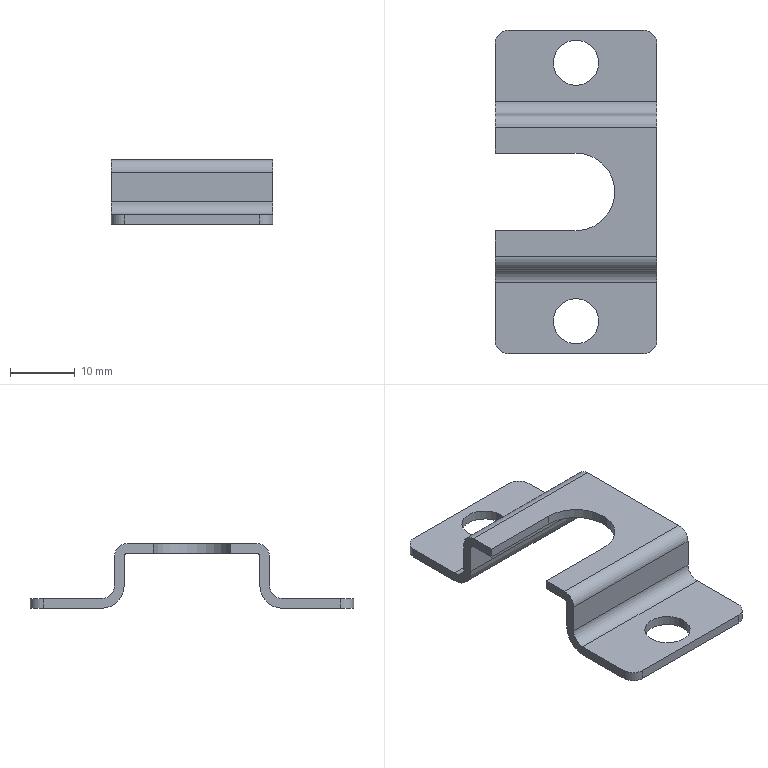Component | SolidWorks | DirectPressureVerticalSeal-1_Fastener-1 | 1 solid | 34 faces | box 25 x 50 x 10 mm | volume 1953 mm3 | cylinder 17 | plane 17 | commonest cylinder face diameters 4 x8 7 x6 1 x2 12 x1
STEP:
#1=CARTESIAN_POINT('',(-11.899,10.507,10.002));
#2=VERTEX_POINT('',#1);
#3=CARTESIAN_POINT('',(-11.624,10.507,10.002));
#4=VERTEX_POINT('',#3);
#5=CARTESIAN_POINT('',(-11.762,10.507,10.002));
#6=DIRECTION('',(-0.,0.,1.));
#7=DIRECTION('',(1.,0.,0.));
#8=AXIS2_PLACEMENT_3D('',#5,#6,#7);
#9=CIRCLE('',#8,0.1378);
#10=EDGE_CURVE('',#2,#4,#9,.T.);
#11=ORIENTED_EDGE('',*,*,#10,.F.);
#12=CARTESIAN_POINT('',(-11.899,10.507,10.061));
#13=VERTEX_POINT('',#12);
#14=CARTESIAN_POINT('',(-11.899,10.507,10.061));
#15=DIRECTION('',(-0.,0.,1.));
#16=VECTOR('',#15,39.37);
#17=LINE('',#14,#16);
#18=EDGE_CURVE('',#2,#13,#17,.T.);
#19=ORIENTED_EDGE('',*,*,#18,.T.);
#20=CARTESIAN_POINT('',(-11.624,10.507,10.061));
#21=VERTEX_POINT('',#20);
#22=CARTESIAN_POINT('',(-11.762,10.507,10.061));
#23=DIRECTION('',(-0.,0.,1.));
#24=DIRECTION('',(1.,0.,0.));
#25=AXIS2_PLACEMENT_3D('',#22,#23,#24);
#26=CIRCLE('',#25,0.1378);
#27=EDGE_CURVE('',#13,#21,#26,.T.);
#28=ORIENTED_EDGE('',*,*,#27,.T.);
#29=CARTESIAN_POINT('',(-11.624,10.507,10.061));
#30=DIRECTION('',(-0.,0.,1.));
#31=VECTOR('',#30,39.37);
#32=LINE('',#29,#31);
#33=EDGE_CURVE('',#4,#21,#32,.T.);
#34=ORIENTED_EDGE('',*,*,#33,.F.);
#35=EDGE_LOOP('',(#11,#19,#28,#34));
#36=FACE_OUTER_BOUND('',#35,.T.);
#37=CARTESIAN_POINT('',(-11.762,10.507,10.061));
#38=DIRECTION('',(-0.,0.,1.));
#39=DIRECTION('',(1.,0.,0.));
#40=AXIS2_PLACEMENT_3D('',#37,#38,#39);
#41=CYLINDRICAL_SURFACE('',#40,0.1378);
#42=ADVANCED_FACE('',(#36),#41,.F.);
#43=CARTESIAN_POINT('',(-11.624,8.932,10.061));
#44=VERTEX_POINT('',#43);
#45=CARTESIAN_POINT('',(-11.899,8.932,10.061));
#46=VERTEX_POINT('',#45);
#47=CARTESIAN_POINT('',(-11.762,8.932,10.061));
#48=DIRECTION('',(0.,-0.,-1.));
#49=DIRECTION('',(0.,1.,0.));
#50=AXIS2_PLACEMENT_3D('',#47,#48,#49);
#51=CIRCLE('',#50,0.1378);
#52=EDGE_CURVE('',#44,#46,#51,.T.);
#53=ORIENTED_EDGE('',*,*,#52,.F.);
#54=CARTESIAN_POINT('',(-11.624,8.932,10.002));
#55=VERTEX_POINT('',#54);
#56=CARTESIAN_POINT('',(-11.624,8.932,10.002));
#57=DIRECTION('',(0.,-0.,-1.));
#58=VECTOR('',#57,39.37);
#59=LINE('',#56,#58);
#60=EDGE_CURVE('',#44,#55,#59,.T.);
#61=ORIENTED_EDGE('',*,*,#60,.T.);
#62=CARTESIAN_POINT('',(-11.899,8.932,10.002));
#63=VERTEX_POINT('',#62);
#64=CARTESIAN_POINT('',(-11.762,8.932,10.002));
#65=DIRECTION('',(0.,-0.,-1.));
#66=DIRECTION('',(-1.,0.,0.));
#67=AXIS2_PLACEMENT_3D('',#64,#65,#66);
#68=CIRCLE('',#67,0.1378);
#69=EDGE_CURVE('',#55,#63,#68,.T.);
#70=ORIENTED_EDGE('',*,*,#69,.T.);
#71=CARTESIAN_POINT('',(-11.899,8.932,10.002));
#72=DIRECTION('',(0.,-0.,-1.));
#73=VECTOR('',#72,39.37);
#74=LINE('',#71,#73);
#75=EDGE_CURVE('',#46,#63,#74,.T.);
#76=ORIENTED_EDGE('',*,*,#75,.F.);
#77=EDGE_LOOP('',(#53,#61,#70,#76));
#78=FACE_OUTER_BOUND('',#77,.T.);
#79=CARTESIAN_POINT('',(-11.762,8.932,10.002));
#80=DIRECTION('',(0.,-0.,-1.));
#81=DIRECTION('',(-1.,0.,0.));
#82=AXIS2_PLACEMENT_3D('',#79,#80,#81);
#83=CYLINDRICAL_SURFACE('',#82,0.1378);
#84=ADVANCED_FACE('',(#78),#83,.F.);
#85=CARTESIAN_POINT('',(-12.254,9.956,10.337));
#86=VERTEX_POINT('',#85);
#87=CARTESIAN_POINT('',(-12.254,10.113,10.337));
#88=VERTEX_POINT('',#87);
#89=CARTESIAN_POINT('',(-12.254,9.168,10.337));
#90=DIRECTION('',(-0.,1.,-0.));
#91=VECTOR('',#90,39.37);
#92=LINE('',#89,#91);
#93=EDGE_CURVE('',#86,#88,#92,.T.);
#94=ORIENTED_EDGE('',*,*,#93,.F.);
#95=CARTESIAN_POINT('',(-12.254,9.956,10.396));
#96=VERTEX_POINT('',#95);
#97=CARTESIAN_POINT('',(-12.254,9.956,10.002));
#98=DIRECTION('',(-0.,0.,1.));
#99=VECTOR('',#98,39.37);
#100=LINE('',#97,#99);
#101=EDGE_CURVE('',#86,#96,#100,.T.);
#102=ORIENTED_EDGE('',*,*,#101,.T.);
#103=CARTESIAN_POINT('',(-12.254,10.113,10.396));
#104=VERTEX_POINT('',#103);
#105=CARTESIAN_POINT('',(-12.254,10.113,10.396));
#106=DIRECTION('',(-0.,1.,-0.));
#107=VECTOR('',#106,39.37);
#108=LINE('',#105,#107);
#109=EDGE_CURVE('',#96,#104,#108,.T.);
#110=ORIENTED_EDGE('',*,*,#109,.T.);
#111=CARTESIAN_POINT('',(-12.254,10.192,10.317));
#112=VERTEX_POINT('',#111);
#113=CARTESIAN_POINT('',(-12.254,10.113,10.317));
#114=DIRECTION('',(1.,0.,0.));
#115=DIRECTION('',(0.,0.,1.));
#116=AXIS2_PLACEMENT_3D('',#113,#114,#115);
#117=CIRCLE('',#116,0.07874);
#118=EDGE_CURVE('',#112,#104,#117,.T.);
#119=ORIENTED_EDGE('',*,*,#118,.F.);
#120=CARTESIAN_POINT('',(-12.254,10.192,10.14));
#121=VERTEX_POINT('',#120);
#122=CARTESIAN_POINT('',(-12.254,10.192,10.14));
#123=DIRECTION('',(-0.,0.,1.));
#124=VECTOR('',#123,39.37);
#125=LINE('',#122,#124);
#126=EDGE_CURVE('',#121,#112,#125,.T.);
#127=ORIENTED_EDGE('',*,*,#126,.F.);
#128=CARTESIAN_POINT('',(-12.254,10.271,10.061));
#129=VERTEX_POINT('',#128);
#130=CARTESIAN_POINT('',(-12.254,10.271,10.14));
#131=DIRECTION('',(-1.,-0.,-0.));
#132=DIRECTION('',(0.,0.,1.));
#133=AXIS2_PLACEMENT_3D('',#130,#131,#132);
#134=CIRCLE('',#133,0.07874);
#135=EDGE_CURVE('',#129,#121,#134,.T.);
#136=ORIENTED_EDGE('',*,*,#135,.F.);
#137=CARTESIAN_POINT('',(-12.254,10.625,10.061));
#138=VERTEX_POINT('',#137);
#139=CARTESIAN_POINT('',(-12.254,9.168,10.061));
#140=DIRECTION('',(0.,-1.,0.));
#141=VECTOR('',#140,39.37);
#142=LINE('',#139,#141);
#143=EDGE_CURVE('',#138,#129,#142,.T.);
#144=ORIENTED_EDGE('',*,*,#143,.F.);
#145=CARTESIAN_POINT('',(-12.254,10.625,10.002));
#146=VERTEX_POINT('',#145);
#147=CARTESIAN_POINT('',(-12.254,10.625,10.14));
#148=DIRECTION('',(-0.,0.,1.));
#149=VECTOR('',#148,39.37);
#150=LINE('',#147,#149);
#151=EDGE_CURVE('',#146,#138,#150,.T.);
#152=ORIENTED_EDGE('',*,*,#151,.F.);
#153=CARTESIAN_POINT('',(-12.254,10.271,10.002));
#154=VERTEX_POINT('',#153);
#155=CARTESIAN_POINT('',(-12.254,9.168,10.002));
#156=DIRECTION('',(-0.,1.,-0.));
#157=VECTOR('',#156,39.37);
#158=LINE('',#155,#157);
#159=EDGE_CURVE('',#154,#146,#158,.T.);
#160=ORIENTED_EDGE('',*,*,#159,.F.);
#161=CARTESIAN_POINT('',(-12.254,10.133,10.14));
#162=VERTEX_POINT('',#161);
#163=CARTESIAN_POINT('',(-12.254,10.271,10.14));
#164=DIRECTION('',(1.,0.,0.));
#165=DIRECTION('',(0.,0.,1.));
#166=AXIS2_PLACEMENT_3D('',#163,#164,#165);
#167=CIRCLE('',#166,0.1378);
#168=EDGE_CURVE('',#162,#154,#167,.T.);
#169=ORIENTED_EDGE('',*,*,#168,.F.);
#170=CARTESIAN_POINT('',(-12.254,10.133,10.317));
#171=VERTEX_POINT('',#170);
#172=CARTESIAN_POINT('',(-12.254,10.133,10.14));
#173=DIRECTION('',(0.,-0.,-1.));
#174=VECTOR('',#173,39.37);
#175=LINE('',#172,#174);
#176=EDGE_CURVE('',#171,#162,#175,.T.);
#177=ORIENTED_EDGE('',*,*,#176,.F.);
#178=CARTESIAN_POINT('',(-12.254,10.113,10.317));
#179=DIRECTION('',(1.,0.,0.));
#180=DIRECTION('',(0.,0.,1.));
#181=AXIS2_PLACEMENT_3D('',#178,#179,#180);
#182=CIRCLE('',#181,0.01969);
#183=EDGE_CURVE('',#171,#88,#182,.T.);
#184=ORIENTED_EDGE('',*,*,#183,.T.);
#185=EDGE_LOOP('',(#94,#102,#110,#119,#127,#136,#144,#152,#160,#169,#177,#184));
#186=FACE_OUTER_BOUND('',#185,.T.);
#187=CARTESIAN_POINT('',(-12.254,9.168,10.14));
#188=DIRECTION('',(1.,0.,0.));
#189=DIRECTION('',(0.,-0.,-1.));
#190=AXIS2_PLACEMENT_3D('',#187,#188,#189);
#191=PLANE('',#190);
#192=ADVANCED_FACE('',(#186),#191,.F.);
#193=ORIENTED_EDGE('',*,*,#109,.F.);
#194=CARTESIAN_POINT('',(-11.762,9.956,10.396));
#195=VERTEX_POINT('',#194);
#196=CARTESIAN_POINT('',(-11.762,9.956,10.396));
#197=DIRECTION('',(-1.,-0.,-0.));
#198=VECTOR('',#197,39.37);
#199=LINE('',#196,#198);
#200=EDGE_CURVE('',#195,#96,#199,.T.);
#201=ORIENTED_EDGE('',*,*,#200,.F.);
#202=CARTESIAN_POINT('',(-11.762,9.483,10.396));
#203=VERTEX_POINT('',#202);
#204=CARTESIAN_POINT('',(-11.762,9.719,10.396));
#205=DIRECTION('',(-0.,0.,1.));
#206=DIRECTION('',(0.,-1.,0.));
#207=AXIS2_PLACEMENT_3D('',#204,#205,#206);
#208=CIRCLE('',#207,0.2362);
#209=EDGE_CURVE('',#203,#195,#208,.T.);
#210=ORIENTED_EDGE('',*,*,#209,.F.);
#211=CARTESIAN_POINT('',(-12.254,9.483,10.396));
#212=VERTEX_POINT('',#211);
#213=CARTESIAN_POINT('',(-12.254,9.483,10.396));
#214=DIRECTION('',(1.,0.,0.));
#215=VECTOR('',#214,39.37);
#216=LINE('',#213,#215);
#217=EDGE_CURVE('',#212,#203,#216,.T.);
#218=ORIENTED_EDGE('',*,*,#217,.F.);
#219=CARTESIAN_POINT('',(-12.254,9.326,10.396));
#220=VERTEX_POINT('',#219);
#221=CARTESIAN_POINT('',(-12.254,10.113,10.396));
#222=DIRECTION('',(-0.,1.,-0.));
#223=VECTOR('',#222,39.37);
#224=LINE('',#221,#223);
#225=EDGE_CURVE('',#220,#212,#224,.T.);
#226=ORIENTED_EDGE('',*,*,#225,.F.);
#227=CARTESIAN_POINT('',(-11.27,9.326,10.396));
#228=VERTEX_POINT('',#227);
#229=CARTESIAN_POINT('',(-11.27,9.326,10.396));
#230=DIRECTION('',(-1.,-0.,-0.));
#231=VECTOR('',#230,39.37);
#232=LINE('',#229,#231);
#233=EDGE_CURVE('',#228,#220,#232,.T.);
#234=ORIENTED_EDGE('',*,*,#233,.F.);
#235=CARTESIAN_POINT('',(-11.27,10.113,10.396));
#236=VERTEX_POINT('',#235);
#237=CARTESIAN_POINT('',(-11.27,10.113,10.396));
#238=DIRECTION('',(0.,-1.,0.));
#239=VECTOR('',#238,39.37);
#240=LINE('',#237,#239);
#241=EDGE_CURVE('',#236,#228,#240,.T.);
#242=ORIENTED_EDGE('',*,*,#241,.F.);
#243=CARTESIAN_POINT('',(-11.27,10.113,10.396));
#244=DIRECTION('',(1.,0.,0.));
#245=VECTOR('',#244,39.37);
#246=LINE('',#243,#245);
#247=EDGE_CURVE('',#104,#236,#246,.T.);
#248=ORIENTED_EDGE('',*,*,#247,.F.);
#249=EDGE_LOOP('',(#193,#201,#210,#218,#226,#234,#242,#248));
#250=FACE_OUTER_BOUND('',#249,.T.);
#251=CARTESIAN_POINT('',(-11.27,10.113,10.396));
#252=DIRECTION('',(0.,-0.,-1.));
#253=DIRECTION('',(-0.,1.,-0.));
#254=AXIS2_PLACEMENT_3D('',#251,#252,#253);
#255=PLANE('',#254);
#256=ADVANCED_FACE('',(#250),#255,.F.);
#257=ORIENTED_EDGE('',*,*,#225,.T.);
#258=CARTESIAN_POINT('',(-12.254,9.483,10.337));
#259=VERTEX_POINT('',#258);
#260=CARTESIAN_POINT('',(-12.254,9.483,10.002));
#261=DIRECTION('',(-0.,0.,1.));
#262=VECTOR('',#261,39.37);
#263=LINE('',#260,#262);
#264=EDGE_CURVE('',#259,#212,#263,.T.);
#265=ORIENTED_EDGE('',*,*,#264,.F.);
#266=CARTESIAN_POINT('',(-12.254,9.326,10.337));
#267=VERTEX_POINT('',#266);
#268=CARTESIAN_POINT('',(-12.254,9.168,10.337));
#269=DIRECTION('',(-0.,1.,-0.));
#270=VECTOR('',#269,39.37);
#271=LINE('',#268,#270);
#272=EDGE_CURVE('',#267,#259,#271,.T.);
#273=ORIENTED_EDGE('',*,*,#272,.F.);
#274=CARTESIAN_POINT('',(-12.254,9.306,10.317));
#275=VERTEX_POINT('',#274);
#276=CARTESIAN_POINT('',(-12.254,9.326,10.317));
#277=DIRECTION('',(1.,0.,0.));
#278=DIRECTION('',(0.,0.,1.));
#279=AXIS2_PLACEMENT_3D('',#276,#277,#278);
#280=CIRCLE('',#279,0.01969);
#281=EDGE_CURVE('',#267,#275,#280,.T.);
#282=ORIENTED_EDGE('',*,*,#281,.T.);
#283=CARTESIAN_POINT('',(-12.254,9.306,10.14));
#284=VERTEX_POINT('',#283);
#285=CARTESIAN_POINT('',(-12.254,9.306,10.14));
#286=DIRECTION('',(-0.,0.,1.));
#287=VECTOR('',#286,39.37);
#288=LINE('',#285,#287);
#289=EDGE_CURVE('',#284,#275,#288,.T.);
#290=ORIENTED_EDGE('',*,*,#289,.F.);
#291=CARTESIAN_POINT('',(-12.254,9.168,10.002));
#292=VERTEX_POINT('',#291);
#293=CARTESIAN_POINT('',(-12.254,9.168,10.14));
#294=DIRECTION('',(1.,0.,0.));
#295=DIRECTION('',(0.,0.,1.));
#296=AXIS2_PLACEMENT_3D('',#293,#294,#295);
#297=CIRCLE('',#296,0.1378);
#298=EDGE_CURVE('',#292,#284,#297,.T.);
#299=ORIENTED_EDGE('',*,*,#298,.F.);
#300=CARTESIAN_POINT('',(-12.254,8.814,10.002));
#301=VERTEX_POINT('',#300);
#302=CARTESIAN_POINT('',(-12.254,9.168,10.002));
#303=DIRECTION('',(-0.,1.,-0.));
#304=VECTOR('',#303,39.37);
#305=LINE('',#302,#304);
#306=EDGE_CURVE('',#301,#292,#305,.T.);
#307=ORIENTED_EDGE('',*,*,#306,.F.);
#308=CARTESIAN_POINT('',(-12.254,8.814,10.061));
#309=VERTEX_POINT('',#308);
#310=CARTESIAN_POINT('',(-12.254,8.814,10.14));
#311=DIRECTION('',(0.,-0.,-1.));
#312=VECTOR('',#311,39.37);
#313=LINE('',#310,#312);
#314=EDGE_CURVE('',#309,#301,#313,.T.);
#315=ORIENTED_EDGE('',*,*,#314,.F.);
#316=CARTESIAN_POINT('',(-12.254,9.168,10.061));
#317=VERTEX_POINT('',#316);
#318=CARTESIAN_POINT('',(-12.254,9.168,10.061));
#319=DIRECTION('',(0.,-1.,0.));
#320=VECTOR('',#319,39.37);
#321=LINE('',#318,#320);
#322=EDGE_CURVE('',#317,#309,#321,.T.);
#323=ORIENTED_EDGE('',*,*,#322,.F.);
#324=CARTESIAN_POINT('',(-12.254,9.247,10.14));
#325=VERTEX_POINT('',#324);
#326=CARTESIAN_POINT('',(-12.254,9.168,10.14));
#327=DIRECTION('',(-1.,-0.,-0.));
#328=DIRECTION('',(0.,0.,1.));
#329=AXIS2_PLACEMENT_3D('',#326,#327,#328);
#330=CIRCLE('',#329,0.07874);
#331=EDGE_CURVE('',#325,#317,#330,.T.);
#332=ORIENTED_EDGE('',*,*,#331,.F.);
#333=CARTESIAN_POINT('',(-12.254,9.247,10.317));
#334=VERTEX_POINT('',#333);
#335=CARTESIAN_POINT('',(-12.254,9.247,10.14));
#336=DIRECTION('',(0.,-0.,-1.));
#337=VECTOR('',#336,39.37);
#338=LINE('',#335,#337);
#339=EDGE_CURVE('',#334,#325,#338,.T.);
#340=ORIENTED_EDGE('',*,*,#339,.F.);
#341=CARTESIAN_POINT('',(-12.254,9.326,10.317));
#342=DIRECTION('',(1.,0.,0.));
#343=DIRECTION('',(0.,0.,1.));
#344=AXIS2_PLACEMENT_3D('',#341,#342,#343);
#345=CIRCLE('',#344,0.07874);
#346=EDGE_CURVE('',#220,#334,#345,.T.);
#347=ORIENTED_EDGE('',*,*,#346,.F.);
#348=EDGE_LOOP('',(#257,#265,#273,#282,#290,#299,#307,#315,#323,#332,#340,#347));
#349=FACE_OUTER_BOUND('',#348,.T.);
#350=CARTESIAN_POINT('',(-12.254,9.168,10.14));
#351=DIRECTION('',(1.,0.,0.));
#352=DIRECTION('',(0.,-0.,-1.));
#353=AXIS2_PLACEMENT_3D('',#350,#351,#352);
#354=PLANE('',#353);
#355=ADVANCED_FACE('',(#349),#354,.F.);
#356=ORIENTED_EDGE('',*,*,#346,.T.);
#357=CARTESIAN_POINT('',(-11.27,9.247,10.317));
#358=VERTEX_POINT('',#357);
#359=CARTESIAN_POINT('',(-11.27,9.247,10.317));
#360=DIRECTION('',(1.,0.,0.));
#361=VECTOR('',#360,39.37);
#362=LINE('',#359,#361);
#363=EDGE_CURVE('',#334,#358,#362,.T.);
#364=ORIENTED_EDGE('',*,*,#363,.T.);
#365=CARTESIAN_POINT('',(-11.27,9.326,10.317));
#366=DIRECTION('',(-1.,-0.,-0.));
#367=DIRECTION('',(0.,0.,1.));
#368=AXIS2_PLACEMENT_3D('',#365,#366,#367);
#369=CIRCLE('',#368,0.07874);
#370=EDGE_CURVE('',#358,#228,#369,.T.);
#371=ORIENTED_EDGE('',*,*,#370,.T.);
#372=ORIENTED_EDGE('',*,*,#233,.T.);
#373=EDGE_LOOP('',(#356,#364,#371,#372));
#374=FACE_OUTER_BOUND('',#373,.T.);
#375=CARTESIAN_POINT('',(-11.27,9.326,10.317));
#376=DIRECTION('',(-1.,-0.,-0.));
#377=DIRECTION('',(0.,0.,1.));
#378=AXIS2_PLACEMENT_3D('',#375,#376,#377);
#379=CYLINDRICAL_SURFACE('',#378,0.07874);
#380=ADVANCED_FACE('',(#374),#379,.T.);
#381=ORIENTED_EDGE('',*,*,#241,.T.);
#382=ORIENTED_EDGE('',*,*,#370,.F.);
#383=CARTESIAN_POINT('',(-11.27,9.247,10.14));
#384=VERTEX_POINT('',#383);
#385=CARTESIAN_POINT('',(-11.27,9.247,10.14));
#386=DIRECTION('',(0.,-0.,-1.));
#387=VECTOR('',#386,39.37);
#388=LINE('',#385,#387);
#389=EDGE_CURVE('',#358,#384,#388,.T.);
#390=ORIENTED_EDGE('',*,*,#389,.T.);
#391=CARTESIAN_POINT('',(-11.27,9.168,10.061));
#392=VERTEX_POINT('',#391);
#393=CARTESIAN_POINT('',(-11.27,9.168,10.14));
#394=DIRECTION('',(-1.,-0.,-0.));
#395=DIRECTION('',(0.,0.,1.));
#396=AXIS2_PLACEMENT_3D('',#393,#394,#395);
#397=CIRCLE('',#396,0.07874);
#398=EDGE_CURVE('',#384,#392,#397,.T.);
#399=ORIENTED_EDGE('',*,*,#398,.T.);
#400=CARTESIAN_POINT('',(-11.27,8.814,10.061));
#401=VERTEX_POINT('',#400);
#402=CARTESIAN_POINT('',(-11.27,9.168,10.061));
#403=DIRECTION('',(0.,-1.,0.));
#404=VECTOR('',#403,39.37);
#405=LINE('',#402,#404);
#406=EDGE_CURVE('',#392,#401,#405,.T.);
#407=ORIENTED_EDGE('',*,*,#406,.T.);
#408=CARTESIAN_POINT('',(-11.27,8.814,10.002));
#409=VERTEX_POINT('',#408);
#410=CARTESIAN_POINT('',(-11.27,8.814,10.002));
#411=DIRECTION('',(-0.,0.,1.));
#412=VECTOR('',#411,39.37);
#413=LINE('',#410,#412);
#414=EDGE_CURVE('',#409,#401,#413,.T.);
#415=ORIENTED_EDGE('',*,*,#414,.F.);
#416=CARTESIAN_POINT('',(-11.27,9.168,10.002));
#417=VERTEX_POINT('',#416);
#418=CARTESIAN_POINT('',(-11.27,9.168,10.002));
#419=DIRECTION('',(-0.,1.,-0.));
#420=VECTOR('',#419,39.37);
#421=LINE('',#418,#420);
#422=EDGE_CURVE('',#409,#417,#421,.T.);
#423=ORIENTED_EDGE('',*,*,#422,.T.);
#424=CARTESIAN_POINT('',(-11.27,9.306,10.14));
#425=VERTEX_POINT('',#424);
#426=CARTESIAN_POINT('',(-11.27,9.168,10.14));
#427=DIRECTION('',(1.,0.,0.));
#428=DIRECTION('',(0.,0.,1.));
#429=AXIS2_PLACEMENT_3D('',#426,#427,#428);
#430=CIRCLE('',#429,0.1378);
#431=EDGE_CURVE('',#417,#425,#430,.T.);
#432=ORIENTED_EDGE('',*,*,#431,.T.);
#433=CARTESIAN_POINT('',(-11.27,9.306,10.317));
#434=VERTEX_POINT('',#433);
#435=CARTESIAN_POINT('',(-11.27,9.306,10.14));
#436=DIRECTION('',(-0.,0.,1.));
#437=VECTOR('',#436,39.37);
#438=LINE('',#435,#437);
#439=EDGE_CURVE('',#425,#434,#438,.T.);
#440=ORIENTED_EDGE('',*,*,#439,.T.);
#441=CARTESIAN_POINT('',(-11.27,9.326,10.337));
#442=VERTEX_POINT('',#441);
#443=CARTESIAN_POINT('',(-11.27,9.326,10.317));
#444=DIRECTION('',(-1.,-0.,-0.));
#445=DIRECTION('',(0.,0.,1.));
#446=AXIS2_PLACEMENT_3D('',#443,#444,#445);
#447=CIRCLE('',#446,0.01969);
#448=EDGE_CURVE('',#434,#442,#447,.T.);
#449=ORIENTED_EDGE('',*,*,#448,.T.);
#450=CARTESIAN_POINT('',(-11.27,10.113,10.337));
#451=VERTEX_POINT('',#450);
#452=CARTESIAN_POINT('',(-11.27,9.168,10.337));
#453=DIRECTION('',(-0.,1.,-0.));
#454=VECTOR('',#453,39.37);
#455=LINE('',#452,#454);
#456=EDGE_CURVE('',#442,#451,#455,.T.);
#457=ORIENTED_EDGE('',*,*,#456,.T.);
#458=CARTESIAN_POINT('',(-11.27,10.133,10.317));
#459=VERTEX_POINT('',#458);
#460=CARTESIAN_POINT('',(-11.27,10.113,10.317));
#461=DIRECTION('',(-1.,-0.,-0.));
#462=DIRECTION('',(0.,0.,1.));
#463=AXIS2_PLACEMENT_3D('',#460,#461,#462);
#464=CIRCLE('',#463,0.01969);
#465=EDGE_CURVE('',#451,#459,#464,.T.);
#466=ORIENTED_EDGE('',*,*,#465,.T.);
#467=CARTESIAN_POINT('',(-11.27,10.133,10.14));
#468=VERTEX_POINT('',#467);
#469=CARTESIAN_POINT('',(-11.27,10.133,10.14));
#470=DIRECTION('',(0.,-0.,-1.));
#471=VECTOR('',#470,39.37);
#472=LINE('',#469,#471);
#473=EDGE_CURVE('',#459,#468,#472,.T.);
#474=ORIENTED_EDGE('',*,*,#473,.T.);
#475=CARTESIAN_POINT('',(-11.27,10.271,10.002));
#476=VERTEX_POINT('',#475);
#477=CARTESIAN_POINT('',(-11.27,10.271,10.14));
#478=DIRECTION('',(1.,0.,0.));
#479=DIRECTION('',(0.,0.,1.));
#480=AXIS2_PLACEMENT_3D('',#477,#478,#479);
#481=CIRCLE('',#480,0.1378);
#482=EDGE_CURVE('',#468,#476,#481,.T.);
#483=ORIENTED_EDGE('',*,*,#482,.T.);
#484=CARTESIAN_POINT('',(-11.27,10.625,10.002));
#485=VERTEX_POINT('',#484);
#486=CARTESIAN_POINT('',(-11.27,9.168,10.002));
#487=DIRECTION('',(-0.,1.,-0.));
#488=VECTOR('',#487,39.37);
#489=LINE('',#486,#488);
#490=EDGE_CURVE('',#476,#485,#489,.T.);
#491=ORIENTED_EDGE('',*,*,#490,.T.);
#492=CARTESIAN_POINT('',(-11.27,10.625,10.061));
#493=VERTEX_POINT('',#492);
#494=CARTESIAN_POINT('',(-11.27,10.625,10.061));
#495=DIRECTION('',(0.,-0.,-1.));
#496=VECTOR('',#495,39.37);
#497=LINE('',#494,#496);
#498=EDGE_CURVE('',#493,#485,#497,.T.);
#499=ORIENTED_EDGE('',*,*,#498,.F.);
#500=CARTESIAN_POINT('',(-11.27,10.271,10.061));
#501=VERTEX_POINT('',#500);
#502=CARTESIAN_POINT('',(-11.27,9.168,10.061));
#503=DIRECTION('',(0.,-1.,0.));
#504=VECTOR('',#503,39.37);
#505=LINE('',#502,#504);
#506=EDGE_CURVE('',#493,#501,#505,.T.);
#507=ORIENTED_EDGE('',*,*,#506,.T.);
#508=CARTESIAN_POINT('',(-11.27,10.192,10.14));
#509=VERTEX_POINT('',#508);
#510=CARTESIAN_POINT('',(-11.27,10.271,10.14));
#511=DIRECTION('',(-1.,-0.,-0.));
#512=DIRECTION('',(0.,0.,1.));
#513=AXIS2_PLACEMENT_3D('',#510,#511,#512);
#514=CIRCLE('',#513,0.07874);
#515=EDGE_CURVE('',#501,#509,#514,.T.);
#516=ORIENTED_EDGE('',*,*,#515,.T.);
#517=CARTESIAN_POINT('',(-11.27,10.192,10.317));
#518=VERTEX_POINT('',#517);
#519=CARTESIAN_POINT('',(-11.27,10.192,10.14));
#520=DIRECTION('',(-0.,0.,1.));
#521=VECTOR('',#520,39.37);
#522=LINE('',#519,#521);
#523=EDGE_CURVE('',#509,#518,#522,.T.);
#524=ORIENTED_EDGE('',*,*,#523,.T.);
#525=CARTESIAN_POINT('',(-11.27,10.113,10.317));
#526=DIRECTION('',(1.,0.,0.));
#527=DIRECTION('',(0.,0.,1.));
#528=AXIS2_PLACEMENT_3D('',#525,#526,#527);
#529=CIRCLE('',#528,0.07874);
#530=EDGE_CURVE('',#518,#236,#529,.T.);
#531=ORIENTED_EDGE('',*,*,#530,.T.);
#532=EDGE_LOOP('',(#381,#382,#390,#399,#407,#415,#423,#432,#440,#449,#457,#466,#474,#483,#491,#499,#507,#516,#524,#531));
#533=FACE_OUTER_BOUND('',#532,.T.);
#534=CARTESIAN_POINT('',(-11.27,9.168,10.14));
#535=DIRECTION('',(1.,0.,0.));
#536=DIRECTION('',(0.,-0.,-1.));
#537=AXIS2_PLACEMENT_3D('',#534,#535,#536);
#538=PLANE('',#537);
#539=ADVANCED_FACE('',(#533),#538,.T.);
#540=ORIENTED_EDGE('',*,*,#118,.T.);
#541=ORIENTED_EDGE('',*,*,#247,.T.);
#542=ORIENTED_EDGE('',*,*,#530,.F.);
#543=CARTESIAN_POINT('',(-11.27,10.192,10.317));
#544=DIRECTION('',(-1.,-0.,-0.));
#545=VECTOR('',#544,39.37);
#546=LINE('',#543,#545);
#547=EDGE_CURVE('',#518,#112,#546,.T.);
#548=ORIENTED_EDGE('',*,*,#547,.T.);
#549=EDGE_LOOP('',(#540,#541,#542,#548));
#550=FACE_OUTER_BOUND('',#549,.T.);
#551=CARTESIAN_POINT('',(-11.27,10.113,10.317));
#552=DIRECTION('',(-1.,-0.,-0.));
#553=DIRECTION('',(0.,0.,1.));
#554=AXIS2_PLACEMENT_3D('',#551,#552,#553);
#555=CYLINDRICAL_SURFACE('',#554,0.07874);
#556=ADVANCED_FACE('',(#550),#555,.T.);
#557=CARTESIAN_POINT('',(-11.762,9.956,10.337));
#558=VERTEX_POINT('',#557);
#559=CARTESIAN_POINT('',(-11.27,9.956,10.337));
#560=DIRECTION('',(1.,0.,0.));
#561=VECTOR('',#560,39.37);
#562=LINE('',#559,#561);
#563=EDGE_CURVE('',#86,#558,#562,.T.);
#564=ORIENTED_EDGE('',*,*,#563,.F.);
#565=ORIENTED_EDGE('',*,*,#93,.T.);
#566=CARTESIAN_POINT('',(-11.27,10.113,10.337));
#567=DIRECTION('',(1.,0.,0.));
#568=VECTOR('',#567,39.37);
#569=LINE('',#566,#568);
#570=EDGE_CURVE('',#88,#451,#569,.T.);
#571=ORIENTED_EDGE('',*,*,#570,.T.);
#572=ORIENTED_EDGE('',*,*,#456,.F.);
#573=CARTESIAN_POINT('',(-11.27,9.326,10.337));
#574=DIRECTION('',(-1.,-0.,-0.));
#575=VECTOR('',#574,39.37);
#576=LINE('',#573,#575);
#577=EDGE_CURVE('',#442,#267,#576,.T.);
#578=ORIENTED_EDGE('',*,*,#577,.T.);
#579=ORIENTED_EDGE('',*,*,#272,.T.);
#580=CARTESIAN_POINT('',(-11.762,9.483,10.337));
#581=VERTEX_POINT('',#580);
#582=CARTESIAN_POINT('',(-11.27,9.483,10.337));
#583=DIRECTION('',(-1.,-0.,-0.));
#584=VECTOR('',#583,39.37);
#585=LINE('',#582,#584);
#586=EDGE_CURVE('',#581,#259,#585,.T.);
#587=ORIENTED_EDGE('',*,*,#586,.F.);
#588=CARTESIAN_POINT('',(-11.762,9.719,10.337));
#589=DIRECTION('',(0.,-0.,-1.));
#590=DIRECTION('',(0.,1.,0.));
#591=AXIS2_PLACEMENT_3D('',#588,#589,#590);
#592=CIRCLE('',#591,0.2362);
#593=EDGE_CURVE('',#558,#581,#592,.T.);
#594=ORIENTED_EDGE('',*,*,#593,.F.);
#595=EDGE_LOOP('',(#564,#565,#571,#572,#578,#579,#587,#594));
#596=FACE_OUTER_BOUND('',#595,.T.);
#597=CARTESIAN_POINT('',(-11.27,10.113,10.337));
#598=DIRECTION('',(0.,-0.,-1.));
#599=DIRECTION('',(-0.,1.,-0.));
#600=AXIS2_PLACEMENT_3D('',#597,#598,#599);
#601=PLANE('',#600);
#602=ADVANCED_FACE('',(#596),#601,.T.);
#603=ORIENTED_EDGE('',*,*,#289,.T.);
#604=CARTESIAN_POINT('',(-11.27,9.306,10.317));
#605=DIRECTION('',(1.,0.,0.));
#606=VECTOR('',#605,39.37);
#607=LINE('',#604,#606);
#608=EDGE_CURVE('',#275,#434,#607,.T.);
#609=ORIENTED_EDGE('',*,*,#608,.T.);
#610=ORIENTED_EDGE('',*,*,#439,.F.);
#611=CARTESIAN_POINT('',(-11.27,9.306,10.14));
#612=DIRECTION('',(-1.,-0.,-0.));
#613=VECTOR('',#612,39.37);
#614=LINE('',#611,#613);
#615=EDGE_CURVE('',#425,#284,#614,.T.);
#616=ORIENTED_EDGE('',*,*,#615,.T.);
#617=EDGE_LOOP('',(#603,#609,#610,#616));
#618=FACE_OUTER_BOUND('',#617,.T.);
#619=CARTESIAN_POINT('',(-11.27,9.306,10.317));
#620=DIRECTION('',(-0.,1.,-0.));
#621=DIRECTION('',(-0.,0.,1.));
#622=AXIS2_PLACEMENT_3D('',#619,#620,#621);
#623=PLANE('',#622);
#624=ADVANCED_FACE('',(#618),#623,.T.);
#625=ORIENTED_EDGE('',*,*,#298,.T.);
#626=ORIENTED_EDGE('',*,*,#615,.F.);
#627=ORIENTED_EDGE('',*,*,#431,.F.);
#628=CARTESIAN_POINT('',(-11.27,9.168,10.002));
#629=DIRECTION('',(-1.,-0.,-0.));
#630=VECTOR('',#629,39.37);
#631=LINE('',#628,#630);
#632=EDGE_CURVE('',#417,#292,#631,.T.);
#633=ORIENTED_EDGE('',*,*,#632,.T.);
#634=EDGE_LOOP('',(#625,#626,#627,#633));
#635=FACE_OUTER_BOUND('',#634,.T.);
#636=CARTESIAN_POINT('',(-11.27,9.168,10.14));
#637=DIRECTION('',(-1.,-0.,-0.));
#638=DIRECTION('',(0.,0.,1.));
#639=AXIS2_PLACEMENT_3D('',#636,#637,#638);
#640=CYLINDRICAL_SURFACE('',#639,0.1378);
#641=ADVANCED_FACE('',(#635),#640,.T.);
#642=CARTESIAN_POINT('',(-11.762,8.932,10.002));
#643=DIRECTION('',(0.,-0.,-1.));
#644=DIRECTION('',(-1.,0.,0.));
#645=AXIS2_PLACEMENT_3D('',#642,#643,#644);
#646=CIRCLE('',#645,0.1378);
#647=EDGE_CURVE('',#63,#55,#646,.T.);
#648=ORIENTED_EDGE('',*,*,#647,.F.);
#649=ORIENTED_EDGE('',*,*,#69,.F.);
#650=EDGE_LOOP('',(#648,#649));
#651=FACE_BOUND('',#650,.T.);
#652=ORIENTED_EDGE('',*,*,#306,.T.);
#653=ORIENTED_EDGE('',*,*,#632,.F.);
#654=ORIENTED_EDGE('',*,*,#422,.F.);
#655=CARTESIAN_POINT('',(-11.348,8.735,10.002));
#656=VERTEX_POINT('',#655);
#657=CARTESIAN_POINT('',(-11.348,8.814,10.002));
#658=DIRECTION('',(0.,-0.,-1.));
#659=DIRECTION('',(1.,0.,0.));
#660=AXIS2_PLACEMENT_3D('',#657,#658,#659);
#661=CIRCLE('',#660,0.07874);
#662=EDGE_CURVE('',#409,#656,#661,.T.);
#663=ORIENTED_EDGE('',*,*,#662,.T.);
#664=CARTESIAN_POINT('',(-12.175,8.735,10.002));
#665=VERTEX_POINT('',#664);
#666=CARTESIAN_POINT('',(-11.27,8.735,10.002));
#667=DIRECTION('',(-1.,-0.,-0.));
#668=VECTOR('',#667,39.37);
#669=LINE('',#666,#668);
#670=EDGE_CURVE('',#656,#665,#669,.T.);
#671=ORIENTED_EDGE('',*,*,#670,.T.);
#672=CARTESIAN_POINT('',(-12.175,8.814,10.002));
#673=DIRECTION('',(0.,-0.,-1.));
#674=DIRECTION('',(-1.,0.,0.));
#675=AXIS2_PLACEMENT_3D('',#672,#673,#674);
#676=CIRCLE('',#675,0.07874);
#677=EDGE_CURVE('',#665,#301,#676,.T.);
#678=ORIENTED_EDGE('',*,*,#677,.T.);
#679=EDGE_LOOP('',(#652,#653,#654,#663,#671,#678));
#680=FACE_OUTER_BOUND('',#679,.T.);
#681=CARTESIAN_POINT('',(-11.27,9.168,10.002));
#682=DIRECTION('',(0.,-0.,-1.));
#683=DIRECTION('',(-0.,1.,-0.));
#684=AXIS2_PLACEMENT_3D('',#681,#682,#683);
#685=PLANE('',#684);
#686=ADVANCED_FACE('',(#651,#680),#685,.T.);
#687=CARTESIAN_POINT('',(-11.762,8.932,10.061));
#688=DIRECTION('',(0.,-0.,-1.));
#689=DIRECTION('',(0.,1.,0.));
#690=AXIS2_PLACEMENT_3D('',#687,#688,#689);
#691=CIRCLE('',#690,0.1378);
#692=EDGE_CURVE('',#46,#44,#691,.T.);
#693=ORIENTED_EDGE('',*,*,#692,.T.);
#694=ORIENTED_EDGE('',*,*,#52,.T.);
#695=EDGE_LOOP('',(#693,#694));
#696=FACE_BOUND('',#695,.T.);
#697=CARTESIAN_POINT('',(-11.348,8.735,10.061));
#698=VERTEX_POINT('',#697);
#699=CARTESIAN_POINT('',(-12.175,8.735,10.061));
#700=VERTEX_POINT('',#699);
#701=CARTESIAN_POINT('',(-11.27,8.735,10.061));
#702=DIRECTION('',(-1.,-0.,-0.));
#703=VECTOR('',#702,39.37);
#704=LINE('',#701,#703);
#705=EDGE_CURVE('',#698,#700,#704,.T.);
#706=ORIENTED_EDGE('',*,*,#705,.F.);
#707=CARTESIAN_POINT('',(-11.348,8.814,10.061));
#708=DIRECTION('',(0.,-0.,-1.));
#709=DIRECTION('',(1.,0.,0.));
#710=AXIS2_PLACEMENT_3D('',#707,#708,#709);
#711=CIRCLE('',#710,0.07874);
#712=EDGE_CURVE('',#401,#698,#711,.T.);
#713=ORIENTED_EDGE('',*,*,#712,.F.);
#714=ORIENTED_EDGE('',*,*,#406,.F.);
#715=CARTESIAN_POINT('',(-11.27,9.168,10.061));
#716=DIRECTION('',(1.,0.,0.));
#717=VECTOR('',#716,39.37);
#718=LINE('',#715,#717);
#719=EDGE_CURVE('',#317,#392,#718,.T.);
#720=ORIENTED_EDGE('',*,*,#719,.F.);
#721=ORIENTED_EDGE('',*,*,#322,.T.);
#722=CARTESIAN_POINT('',(-12.175,8.814,10.061));
#723=DIRECTION('',(0.,-0.,-1.));
#724=DIRECTION('',(-1.,0.,0.));
#725=AXIS2_PLACEMENT_3D('',#722,#723,#724);
#726=CIRCLE('',#725,0.07874);
#727=EDGE_CURVE('',#700,#309,#726,.T.);
#728=ORIENTED_EDGE('',*,*,#727,.F.);
#729=EDGE_LOOP('',(#706,#713,#714,#720,#721,#728));
#730=FACE_OUTER_BOUND('',#729,.T.);
#731=CARTESIAN_POINT('',(-11.27,9.168,10.061));
#732=DIRECTION('',(0.,-0.,-1.));
#733=DIRECTION('',(-0.,1.,-0.));
#734=AXIS2_PLACEMENT_3D('',#731,#732,#733);
#735=PLANE('',#734);
#736=ADVANCED_FACE('',(#696,#730),#735,.F.);
#737=ORIENTED_EDGE('',*,*,#398,.F.);
#738=CARTESIAN_POINT('',(-11.27,9.247,10.14));
#739=DIRECTION('',(1.,0.,0.));
#740=VECTOR('',#739,39.37);
#741=LINE('',#738,#740);
#742=EDGE_CURVE('',#325,#384,#741,.T.);
#743=ORIENTED_EDGE('',*,*,#742,.F.);
#744=ORIENTED_EDGE('',*,*,#331,.T.);
#745=ORIENTED_EDGE('',*,*,#719,.T.);
#746=EDGE_LOOP('',(#737,#743,#744,#745));
#747=FACE_OUTER_BOUND('',#746,.T.);
#748=CARTESIAN_POINT('',(-11.27,9.168,10.14));
#749=DIRECTION('',(-1.,-0.,-0.));
#750=DIRECTION('',(0.,0.,1.));
#751=AXIS2_PLACEMENT_3D('',#748,#749,#750);
#752=CYLINDRICAL_SURFACE('',#751,0.07874);
#753=ADVANCED_FACE('',(#747),#752,.F.);
#754=ORIENTED_EDGE('',*,*,#389,.F.);
#755=ORIENTED_EDGE('',*,*,#363,.F.);
#756=ORIENTED_EDGE('',*,*,#339,.T.);
#757=ORIENTED_EDGE('',*,*,#742,.T.);
#758=EDGE_LOOP('',(#754,#755,#756,#757));
#759=FACE_OUTER_BOUND('',#758,.T.);
#760=CARTESIAN_POINT('',(-11.27,9.247,10.317));
#761=DIRECTION('',(-0.,1.,-0.));
#762=DIRECTION('',(-0.,0.,1.));
#763=AXIS2_PLACEMENT_3D('',#760,#761,#762);
#764=PLANE('',#763);
#765=ADVANCED_FACE('',(#759),#764,.F.);
#766=ORIENTED_EDGE('',*,*,#523,.F.);
#767=CARTESIAN_POINT('',(-11.27,10.192,10.14));
#768=DIRECTION('',(1.,0.,0.));
#769=VECTOR('',#768,39.37);
#770=LINE('',#767,#769);
#771=EDGE_CURVE('',#121,#509,#770,.T.);
#772=ORIENTED_EDGE('',*,*,#771,.F.);
#773=ORIENTED_EDGE('',*,*,#126,.T.);
#774=ORIENTED_EDGE('',*,*,#547,.F.);
#775=EDGE_LOOP('',(#766,#772,#773,#774));
#776=FACE_OUTER_BOUND('',#775,.T.);
#777=CARTESIAN_POINT('',(-11.27,10.192,10.14));
#778=DIRECTION('',(0.,-1.,0.));
#779=DIRECTION('',(0.,-0.,-1.));
#780=AXIS2_PLACEMENT_3D('',#777,#778,#779);
#781=PLANE('',#780);
#782=ADVANCED_FACE('',(#776),#781,.F.);
#783=ORIENTED_EDGE('',*,*,#515,.F.);
#784=CARTESIAN_POINT('',(-11.27,10.271,10.061));
#785=DIRECTION('',(1.,0.,0.));
#786=VECTOR('',#785,39.37);
#787=LINE('',#784,#786);
#788=EDGE_CURVE('',#129,#501,#787,.T.);
#789=ORIENTED_EDGE('',*,*,#788,.F.);
#790=ORIENTED_EDGE('',*,*,#135,.T.);
#791=ORIENTED_EDGE('',*,*,#771,.T.);
#792=EDGE_LOOP('',(#783,#789,#790,#791));
#793=FACE_OUTER_BOUND('',#792,.T.);
#794=CARTESIAN_POINT('',(-11.27,10.271,10.14));
#795=DIRECTION('',(-1.,-0.,-0.));
#796=DIRECTION('',(0.,0.,1.));
#797=AXIS2_PLACEMENT_3D('',#794,#795,#796);
#798=CYLINDRICAL_SURFACE('',#797,0.07874);
#799=ADVANCED_FACE('',(#793),#798,.F.);
#800=CARTESIAN_POINT('',(-11.762,10.507,10.061));
#801=DIRECTION('',(-0.,0.,1.));
#802=DIRECTION('',(1.,0.,0.));
#803=AXIS2_PLACEMENT_3D('',#800,#801,#802);
#804=CIRCLE('',#803,0.1378);
#805=EDGE_CURVE('',#21,#13,#804,.T.);
#806=ORIENTED_EDGE('',*,*,#805,.F.);
#807=ORIENTED_EDGE('',*,*,#27,.F.);
#808=EDGE_LOOP('',(#806,#807));
#809=FACE_BOUND('',#808,.T.);
#810=ORIENTED_EDGE('',*,*,#143,.T.);
#811=ORIENTED_EDGE('',*,*,#788,.T.);
#812=ORIENTED_EDGE('',*,*,#506,.F.);
#813=CARTESIAN_POINT('',(-11.348,10.704,10.061));
#814=VERTEX_POINT('',#813);
#815=CARTESIAN_POINT('',(-11.348,10.625,10.061));
#816=DIRECTION('',(0.,-0.,-1.));
#817=DIRECTION('',(-1.,0.,0.));
#818=AXIS2_PLACEMENT_3D('',#815,#816,#817);
#819=CIRCLE('',#818,0.07874);
#820=EDGE_CURVE('',#814,#493,#819,.T.);
#821=ORIENTED_EDGE('',*,*,#820,.F.);
#822=CARTESIAN_POINT('',(-12.175,10.704,10.061));
#823=VERTEX_POINT('',#822);
#824=CARTESIAN_POINT('',(-11.27,10.704,10.061));
#825=DIRECTION('',(1.,0.,0.));
#826=VECTOR('',#825,39.37);
#827=LINE('',#824,#826);
#828=EDGE_CURVE('',#823,#814,#827,.T.);
#829=ORIENTED_EDGE('',*,*,#828,.F.);
#830=CARTESIAN_POINT('',(-12.175,10.625,10.061));
#831=DIRECTION('',(0.,-0.,-1.));
#832=DIRECTION('',(1.,0.,0.));
#833=AXIS2_PLACEMENT_3D('',#830,#831,#832);
#834=CIRCLE('',#833,0.07874);
#835=EDGE_CURVE('',#138,#823,#834,.T.);
#836=ORIENTED_EDGE('',*,*,#835,.F.);
#837=EDGE_LOOP('',(#810,#811,#812,#821,#829,#836));
#838=FACE_OUTER_BOUND('',#837,.T.);
#839=CARTESIAN_POINT('',(-11.27,10.704,10.061));
#840=DIRECTION('',(0.,-0.,-1.));
#841=DIRECTION('',(-0.,1.,-0.));
#842=AXIS2_PLACEMENT_3D('',#839,#840,#841);
#843=PLANE('',#842);
#844=ADVANCED_FACE('',(#809,#838),#843,.F.);
#845=CARTESIAN_POINT('',(-11.762,10.507,10.002));
#846=DIRECTION('',(-0.,0.,1.));
#847=DIRECTION('',(1.,0.,0.));
#848=AXIS2_PLACEMENT_3D('',#845,#846,#847);
#849=CIRCLE('',#848,0.1378);
#850=EDGE_CURVE('',#4,#2,#849,.T.);
#851=ORIENTED_EDGE('',*,*,#850,.T.);
#852=ORIENTED_EDGE('',*,*,#10,.T.);
#853=EDGE_LOOP('',(#851,#852));
#854=FACE_BOUND('',#853,.T.);
#855=CARTESIAN_POINT('',(-12.175,10.704,10.002));
#856=VERTEX_POINT('',#855);
#857=CARTESIAN_POINT('',(-11.348,10.704,10.002));
#858=VERTEX_POINT('',#857);
#859=CARTESIAN_POINT('',(-11.27,10.704,10.002));
#860=DIRECTION('',(1.,0.,0.));
#861=VECTOR('',#860,39.37);
#862=LINE('',#859,#861);
#863=EDGE_CURVE('',#856,#858,#862,.T.);
#864=ORIENTED_EDGE('',*,*,#863,.T.);
#865=CARTESIAN_POINT('',(-11.348,10.625,10.002));
#866=DIRECTION('',(0.,-0.,-1.));
#867=DIRECTION('',(-1.,0.,0.));
#868=AXIS2_PLACEMENT_3D('',#865,#866,#867);
#869=CIRCLE('',#868,0.07874);
#870=EDGE_CURVE('',#858,#485,#869,.T.);
#871=ORIENTED_EDGE('',*,*,#870,.T.);
#872=ORIENTED_EDGE('',*,*,#490,.F.);
#873=CARTESIAN_POINT('',(-11.27,10.271,10.002));
#874=DIRECTION('',(-1.,-0.,-0.));
#875=VECTOR('',#874,39.37);
#876=LINE('',#873,#875);
#877=EDGE_CURVE('',#476,#154,#876,.T.);
#878=ORIENTED_EDGE('',*,*,#877,.T.);
#879=ORIENTED_EDGE('',*,*,#159,.T.);
#880=CARTESIAN_POINT('',(-12.175,10.625,10.002));
#881=DIRECTION('',(0.,-0.,-1.));
#882=DIRECTION('',(1.,0.,0.));
#883=AXIS2_PLACEMENT_3D('',#880,#881,#882);
#884=CIRCLE('',#883,0.07874);
#885=EDGE_CURVE('',#146,#856,#884,.T.);
#886=ORIENTED_EDGE('',*,*,#885,.T.);
#887=EDGE_LOOP('',(#864,#871,#872,#878,#879,#886));
#888=FACE_OUTER_BOUND('',#887,.T.);
#889=CARTESIAN_POINT('',(-11.27,10.704,10.002));
#890=DIRECTION('',(0.,-0.,-1.));
#891=DIRECTION('',(-0.,1.,-0.));
#892=AXIS2_PLACEMENT_3D('',#889,#890,#891);
#893=PLANE('',#892);
#894=ADVANCED_FACE('',(#854,#888),#893,.T.);
#895=ORIENTED_EDGE('',*,*,#168,.T.);
#896=ORIENTED_EDGE('',*,*,#877,.F.);
#897=ORIENTED_EDGE('',*,*,#482,.F.);
#898=CARTESIAN_POINT('',(-11.27,10.133,10.14));
#899=DIRECTION('',(-1.,-0.,-0.));
#900=VECTOR('',#899,39.37);
#901=LINE('',#898,#900);
#902=EDGE_CURVE('',#468,#162,#901,.T.);
#903=ORIENTED_EDGE('',*,*,#902,.T.);
#904=EDGE_LOOP('',(#895,#896,#897,#903));
#905=FACE_OUTER_BOUND('',#904,.T.);
#906=CARTESIAN_POINT('',(-11.27,10.271,10.14));
#907=DIRECTION('',(-1.,-0.,-0.));
#908=DIRECTION('',(0.,0.,1.));
#909=AXIS2_PLACEMENT_3D('',#906,#907,#908);
#910=CYLINDRICAL_SURFACE('',#909,0.1378);
#911=ADVANCED_FACE('',(#905),#910,.T.);
#912=ORIENTED_EDGE('',*,*,#176,.T.);
#913=ORIENTED_EDGE('',*,*,#902,.F.);
#914=ORIENTED_EDGE('',*,*,#473,.F.);
#915=CARTESIAN_POINT('',(-11.27,10.133,10.317));
#916=DIRECTION('',(-1.,-0.,-0.));
#917=VECTOR('',#916,39.37);
#918=LINE('',#915,#917);
#919=EDGE_CURVE('',#459,#171,#918,.T.);
#920=ORIENTED_EDGE('',*,*,#919,.T.);
#921=EDGE_LOOP('',(#912,#913,#914,#920));
#922=FACE_OUTER_BOUND('',#921,.T.);
#923=CARTESIAN_POINT('',(-11.27,10.133,10.14));
#924=DIRECTION('',(0.,-1.,0.));
#925=DIRECTION('',(0.,-0.,-1.));
#926=AXIS2_PLACEMENT_3D('',#923,#924,#925);
#927=PLANE('',#926);
#928=ADVANCED_FACE('',(#922),#927,.T.);
#929=ORIENTED_EDGE('',*,*,#465,.F.);
#930=ORIENTED_EDGE('',*,*,#570,.F.);
#931=ORIENTED_EDGE('',*,*,#183,.F.);
#932=ORIENTED_EDGE('',*,*,#919,.F.);
#933=EDGE_LOOP('',(#929,#930,#931,#932));
#934=FACE_OUTER_BOUND('',#933,.T.);
#935=CARTESIAN_POINT('',(-11.27,10.113,10.317));
#936=DIRECTION('',(-1.,-0.,-0.));
#937=DIRECTION('',(0.,0.,1.));
#938=AXIS2_PLACEMENT_3D('',#935,#936,#937);
#939=CYLINDRICAL_SURFACE('',#938,0.01969);
#940=ADVANCED_FACE('',(#934),#939,.F.);
#941=ORIENTED_EDGE('',*,*,#448,.F.);
#942=ORIENTED_EDGE('',*,*,#608,.F.);
#943=ORIENTED_EDGE('',*,*,#281,.F.);
#944=ORIENTED_EDGE('',*,*,#577,.F.);
#945=EDGE_LOOP('',(#941,#942,#943,#944));
#946=FACE_OUTER_BOUND('',#945,.T.);
#947=CARTESIAN_POINT('',(-11.27,9.326,10.317));
#948=DIRECTION('',(-1.,-0.,-0.));
#949=DIRECTION('',(0.,0.,1.));
#950=AXIS2_PLACEMENT_3D('',#947,#948,#949);
#951=CYLINDRICAL_SURFACE('',#950,0.01969);
#952=ADVANCED_FACE('',(#946),#951,.F.);
#953=ORIENTED_EDGE('',*,*,#677,.F.);
#954=CARTESIAN_POINT('',(-12.175,8.735,10.14));
#955=DIRECTION('',(-0.,0.,1.));
#956=VECTOR('',#955,39.37);
#957=LINE('',#954,#956);
#958=EDGE_CURVE('',#665,#700,#957,.T.);
#959=ORIENTED_EDGE('',*,*,#958,.T.);
#960=ORIENTED_EDGE('',*,*,#727,.T.);
#961=ORIENTED_EDGE('',*,*,#314,.T.);
#962=EDGE_LOOP('',(#953,#959,#960,#961));
#963=FACE_OUTER_BOUND('',#962,.T.);
#964=CARTESIAN_POINT('',(-12.175,8.814,10.14));
#965=DIRECTION('',(0.,-0.,-1.));
#966=DIRECTION('',(-1.,0.,0.));
#967=AXIS2_PLACEMENT_3D('',#964,#965,#966);
#968=CYLINDRICAL_SURFACE('',#967,0.07874);
#969=ADVANCED_FACE('',(#963),#968,.T.);
#970=ORIENTED_EDGE('',*,*,#705,.T.);
#971=ORIENTED_EDGE('',*,*,#958,.F.);
#972=ORIENTED_EDGE('',*,*,#670,.F.);
#973=CARTESIAN_POINT('',(-11.348,8.735,10.002));
#974=DIRECTION('',(-0.,0.,1.));
#975=VECTOR('',#974,39.37);
#976=LINE('',#973,#975);
#977=EDGE_CURVE('',#656,#698,#976,.T.);
#978=ORIENTED_EDGE('',*,*,#977,.T.);
#979=EDGE_LOOP('',(#970,#971,#972,#978));
#980=FACE_OUTER_BOUND('',#979,.T.);
#981=CARTESIAN_POINT('',(-11.27,8.735,10.002));
#982=DIRECTION('',(0.,-1.,0.));
#983=DIRECTION('',(-1.,-0.,-0.));
#984=AXIS2_PLACEMENT_3D('',#981,#982,#983);
#985=PLANE('',#984);
#986=ADVANCED_FACE('',(#980),#985,.T.);
#987=ORIENTED_EDGE('',*,*,#662,.F.);
#988=ORIENTED_EDGE('',*,*,#414,.T.);
#989=ORIENTED_EDGE('',*,*,#712,.T.);
#990=ORIENTED_EDGE('',*,*,#977,.F.);
#991=EDGE_LOOP('',(#987,#988,#989,#990));
#992=FACE_OUTER_BOUND('',#991,.T.);
#993=CARTESIAN_POINT('',(-11.348,8.814,10.002));
#994=DIRECTION('',(-0.,0.,1.));
#995=DIRECTION('',(1.,0.,0.));
#996=AXIS2_PLACEMENT_3D('',#993,#994,#995);
#997=CYLINDRICAL_SURFACE('',#996,0.07874);
#998=ADVANCED_FACE('',(#992),#997,.T.);
#999=ORIENTED_EDGE('',*,*,#835,.T.);
#1000=CARTESIAN_POINT('',(-12.175,10.704,10.14));
#1001=DIRECTION('',(0.,-0.,-1.));
#1002=VECTOR('',#1001,39.37);
#1003=LINE('',#1000,#1002);
#1004=EDGE_CURVE('',#823,#856,#1003,.T.);
#1005=ORIENTED_EDGE('',*,*,#1004,.T.);
#1006=ORIENTED_EDGE('',*,*,#885,.F.);
#1007=ORIENTED_EDGE('',*,*,#151,.T.);
#1008=EDGE_LOOP('',(#999,#1005,#1006,#1007));
#1009=FACE_OUTER_BOUND('',#1008,.T.);
#1010=CARTESIAN_POINT('',(-12.175,10.625,10.14));
#1011=DIRECTION('',(-0.,0.,1.));
#1012=DIRECTION('',(1.,0.,0.));
#1013=AXIS2_PLACEMENT_3D('',#1010,#1011,#1012);
#1014=CYLINDRICAL_SURFACE('',#1013,0.07874);
#1015=ADVANCED_FACE('',(#1009),#1014,.T.);
#1016=ORIENTED_EDGE('',*,*,#820,.T.);
#1017=ORIENTED_EDGE('',*,*,#498,.T.);
#1018=ORIENTED_EDGE('',*,*,#870,.F.);
#1019=CARTESIAN_POINT('',(-11.348,10.704,10.061));
#1020=DIRECTION('',(-0.,0.,1.));
#1021=VECTOR('',#1020,39.37);
#1022=LINE('',#1019,#1021);
#1023=EDGE_CURVE('',#858,#814,#1022,.T.);
#1024=ORIENTED_EDGE('',*,*,#1023,.T.);
#1025=EDGE_LOOP('',(#1016,#1017,#1018,#1024));
#1026=FACE_OUTER_BOUND('',#1025,.T.);
#1027=CARTESIAN_POINT('',(-11.348,10.625,10.061));
#1028=DIRECTION('',(0.,-0.,-1.));
#1029=DIRECTION('',(-1.,0.,0.));
#1030=AXIS2_PLACEMENT_3D('',#1027,#1028,#1029);
#1031=CYLINDRICAL_SURFACE('',#1030,0.07874);
#1032=ADVANCED_FACE('',(#1026),#1031,.T.);
#1033=ORIENTED_EDGE('',*,*,#863,.F.);
#1034=ORIENTED_EDGE('',*,*,#1004,.F.);
#1035=ORIENTED_EDGE('',*,*,#828,.T.);
#1036=ORIENTED_EDGE('',*,*,#1023,.F.);
#1037=EDGE_LOOP('',(#1033,#1034,#1035,#1036));
#1038=FACE_OUTER_BOUND('',#1037,.T.);
#1039=CARTESIAN_POINT('',(-11.27,10.704,10.061));
#1040=DIRECTION('',(-0.,1.,-0.));
#1041=DIRECTION('',(1.,0.,0.));
#1042=AXIS2_PLACEMENT_3D('',#1039,#1040,#1041);
#1043=PLANE('',#1042);
#1044=ADVANCED_FACE('',(#1038),#1043,.T.);
#1045=ORIENTED_EDGE('',*,*,#563,.T.);
#1046=CARTESIAN_POINT('',(-11.762,9.956,10.002));
#1047=DIRECTION('',(-0.,0.,1.));
#1048=VECTOR('',#1047,39.37);
#1049=LINE('',#1046,#1048);
#1050=EDGE_CURVE('',#558,#195,#1049,.T.);
#1051=ORIENTED_EDGE('',*,*,#1050,.T.);
#1052=ORIENTED_EDGE('',*,*,#200,.T.);
#1053=ORIENTED_EDGE('',*,*,#101,.F.);
#1054=EDGE_LOOP('',(#1045,#1051,#1052,#1053));
#1055=FACE_OUTER_BOUND('',#1054,.T.);
#1056=CARTESIAN_POINT('',(-11.762,9.956,10.002));
#1057=DIRECTION('',(-0.,1.,-0.));
#1058=DIRECTION('',(1.,0.,0.));
#1059=AXIS2_PLACEMENT_3D('',#1056,#1057,#1058);
#1060=PLANE('',#1059);
#1061=ADVANCED_FACE('',(#1055),#1060,.F.);
#1062=ORIENTED_EDGE('',*,*,#593,.T.);
#1063=CARTESIAN_POINT('',(-11.762,9.483,10.002));
#1064=DIRECTION('',(-0.,0.,1.));
#1065=VECTOR('',#1064,39.37);
#1066=LINE('',#1063,#1065);
#1067=EDGE_CURVE('',#581,#203,#1066,.T.);
#1068=ORIENTED_EDGE('',*,*,#1067,.T.);
#1069=ORIENTED_EDGE('',*,*,#209,.T.);
#1070=ORIENTED_EDGE('',*,*,#1050,.F.);
#1071=EDGE_LOOP('',(#1062,#1068,#1069,#1070));
#1072=FACE_OUTER_BOUND('',#1071,.T.);
#1073=CARTESIAN_POINT('',(-11.762,9.719,10.002));
#1074=DIRECTION('',(-0.,0.,1.));
#1075=DIRECTION('',(0.,-1.,0.));
#1076=AXIS2_PLACEMENT_3D('',#1073,#1074,#1075);
#1077=CYLINDRICAL_SURFACE('',#1076,0.2362);
#1078=ADVANCED_FACE('',(#1072),#1077,.F.);
#1079=ORIENTED_EDGE('',*,*,#586,.T.);
#1080=ORIENTED_EDGE('',*,*,#264,.T.);
#1081=ORIENTED_EDGE('',*,*,#217,.T.);
#1082=ORIENTED_EDGE('',*,*,#1067,.F.);
#1083=EDGE_LOOP('',(#1079,#1080,#1081,#1082));
#1084=FACE_OUTER_BOUND('',#1083,.T.);
#1085=CARTESIAN_POINT('',(-12.254,9.483,10.002));
#1086=DIRECTION('',(0.,-1.,0.));
#1087=DIRECTION('',(0.,-0.,-1.));
#1088=AXIS2_PLACEMENT_3D('',#1085,#1086,#1087);
#1089=PLANE('',#1088);
#1090=ADVANCED_FACE('',(#1084),#1089,.F.);
#1091=ORIENTED_EDGE('',*,*,#60,.F.);
#1092=ORIENTED_EDGE('',*,*,#692,.F.);
#1093=ORIENTED_EDGE('',*,*,#75,.T.);
#1094=ORIENTED_EDGE('',*,*,#647,.T.);
#1095=EDGE_LOOP('',(#1091,#1092,#1093,#1094));
#1096=FACE_OUTER_BOUND('',#1095,.T.);
#1097=CARTESIAN_POINT('',(-11.762,8.932,10.002));
#1098=DIRECTION('',(0.,-0.,-1.));
#1099=DIRECTION('',(-1.,0.,0.));
#1100=AXIS2_PLACEMENT_3D('',#1097,#1098,#1099);
#1101=CYLINDRICAL_SURFACE('',#1100,0.1378);
#1102=ADVANCED_FACE('',(#1096),#1101,.F.);
#1103=ORIENTED_EDGE('',*,*,#18,.F.);
#1104=ORIENTED_EDGE('',*,*,#850,.F.);
#1105=ORIENTED_EDGE('',*,*,#33,.T.);
#1106=ORIENTED_EDGE('',*,*,#805,.T.);
#1107=EDGE_LOOP('',(#1103,#1104,#1105,#1106));
#1108=FACE_OUTER_BOUND('',#1107,.T.);
#1109=CARTESIAN_POINT('',(-11.762,10.507,10.061));
#1110=DIRECTION('',(-0.,0.,1.));
#1111=DIRECTION('',(1.,0.,0.));
#1112=AXIS2_PLACEMENT_3D('',#1109,#1110,#1111);
#1113=CYLINDRICAL_SURFACE('',#1112,0.1378);
#1114=ADVANCED_FACE('',(#1108),#1113,.F.);
#1115=CLOSED_SHELL('',(#42,#84,#192,#256,#355,#380,#539,#556,#602,#624,#641,#686,#736,#753,#765,#782,#799,#844,#894,#911,#928,#940,#952,#969,#986,#998,#1015,#1032,#1044,#1061,#1078,#1090,#1102,#1114));
#1116=MANIFOLD_SOLID_BREP('',#1115);
#1117=CARTESIAN_POINT('',(0.,0.,0.));
#1118=DIRECTION('',(0.,0.,1.));
#1119=DIRECTION('',(1.,0.,0.));
#1120=AXIS2_PLACEMENT_3D('',#1117,#1118,#1119);
#1121=(LENGTH_UNIT()NAMED_UNIT(*)SI_UNIT($,.METRE.));
#1122=LENGTH_MEASURE_WITH_UNIT(LENGTH_MEASURE(0.0254),#1121);
#1123=DIMENSIONAL_EXPONENTS(1.,0.,0.,0.,0.,0.,0.);
#1124=(CONVERSION_BASED_UNIT('',#1122)LENGTH_UNIT()NAMED_UNIT(#1123));
#1125=UNCERTAINTY_MEASURE_WITH_UNIT(LENGTH_MEASURE(0.00001),#1124,'','');
#1126=(NAMED_UNIT(*)PLANE_ANGLE_UNIT()SI_UNIT($,.RADIAN.));
#1127=(NAMED_UNIT(*)SI_UNIT($,.STERADIAN.)SOLID_ANGLE_UNIT());
#1128=(GEOMETRIC_REPRESENTATION_CONTEXT(3)GLOBAL_UNCERTAINTY_ASSIGNED_CONTEXT((#1125))GLOBAL_UNIT_ASSIGNED_CONTEXT((#1124,#1126,#1127))REPRESENTATION_CONTEXT('',''));
#1129=ADVANCED_BREP_SHAPE_REPRESENTATION('',(#1116,#1120),#1128);
#1130=COLOUR_RGB('',0.7922,0.8196,0.9333);
#1131=FILL_AREA_STYLE_COLOUR('',#1130);
#1132=FILL_AREA_STYLE('',(#1131));
#1133=SURFACE_STYLE_FILL_AREA(#1132);
#1134=SURFACE_SIDE_STYLE('',(#1133));
#1135=SURFACE_STYLE_USAGE(.BOTH.,#1134);
#1136=PRESENTATION_STYLE_ASSIGNMENT((#1135));
#1137=STYLED_ITEM('',(#1136),#1116);
#1138=PRESENTATION_LAYER_ASSIGNMENT('','',(#1137));
#1139=(LENGTH_UNIT()NAMED_UNIT(*)SI_UNIT($,.METRE.));
#1140=LENGTH_MEASURE_WITH_UNIT(LENGTH_MEASURE(0.0254),#1139);
#1141=DIMENSIONAL_EXPONENTS(1.,0.,0.,0.,0.,0.,0.);
#1142=(CONVERSION_BASED_UNIT('',#1140)LENGTH_UNIT()NAMED_UNIT(#1141));
#1143=UNCERTAINTY_MEASURE_WITH_UNIT(LENGTH_MEASURE(0.00001),#1142,'','');
#1144=(NAMED_UNIT(*)PLANE_ANGLE_UNIT()SI_UNIT($,.RADIAN.));
#1145=(NAMED_UNIT(*)SI_UNIT($,.STERADIAN.)SOLID_ANGLE_UNIT());
#1146=(GEOMETRIC_REPRESENTATION_CONTEXT(3)GLOBAL_UNCERTAINTY_ASSIGNED_CONTEXT((#1143))GLOBAL_UNIT_ASSIGNED_CONTEXT((#1142,#1144,#1145))REPRESENTATION_CONTEXT('',''));
#1147=MECHANICAL_DESIGN_GEOMETRIC_PRESENTATION_REPRESENTATION('',(#1137),#1146);